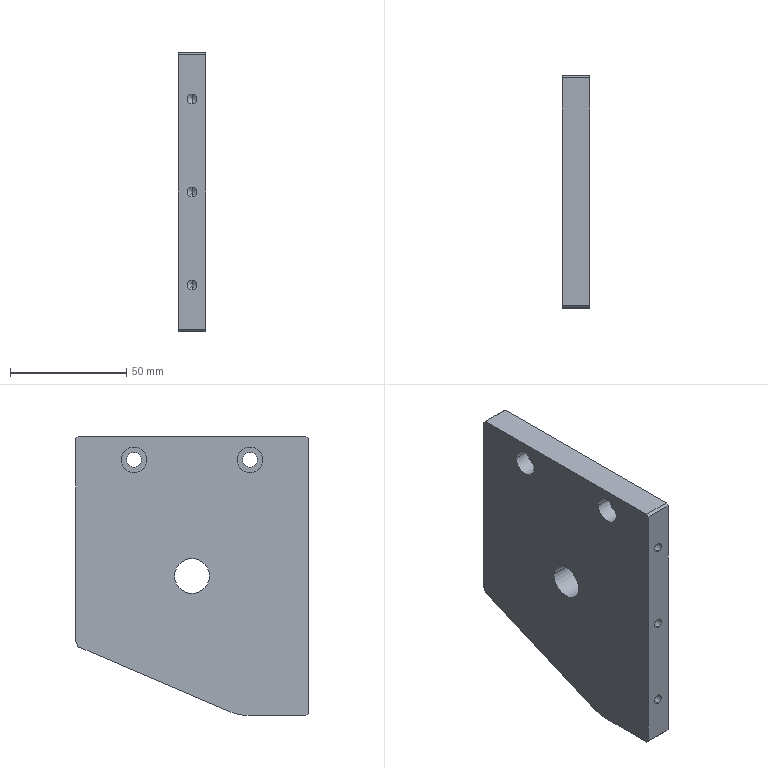Component | SolidWorks | V1ZHXTZ-AxisConnectionPlateReinforcementRibSB1-1 | 1 solid | 36 faces | box 12 x 100 x 120 mm | volume 126870 mm3 | cylinder 17 | plane 13 | cone 6 | commonest cylinder face diameters 4.2 x6 11 x4 6.4 x4 15 x2 40 x1
build123d program:
from build123d import *
from OCP.BRepFilletAPI import BRepFilletAPI_MakeChamfer

# Parameters (mm, degrees)
SKETCH1_W                                         = 120
SKETCH1_H                                         = 100
BOSS_EXTRUDE1_DEPTH                               = 6
CHAMFER1_SIZE                                     = 70
CHAMFER1_SIZE2                                    = 30
M5_TAPPED_HOLE2_D                                 = 4.2
M5_TAPPED_HOLE2_DEPTH                             = 17.4
M5_TAPPED_HOLE2_TIP                               = 1.262
HOLE_SIZE_ACCORDING_TO_TYPE_2_FOR_HEX_D           = 6.4
HOLE_SIZE_ACCORDING_TO_TYPE_2_FOR_HEX_DEPTH       = 18
HOLE_SIZE_ACCORDING_TO_TYPE_2_FOR_HEX_CBORE_D     = 11
HOLE_SIZE_ACCORDING_TO_TYPE_2_FOR_HEX_CBORE_DEPTH = 6.8
HOLE_SIZE_ACCORDING_TO_TYPE_2_FOR_HEX_TIP         = 1.923
CHAMFER2_SIZE                                     = 1
CHAMFER2_SIZE2                                    = 1.904
FILLET1_R                                         = 20
CUT_EXTRUDE1_REACH                                = 81.019
SKETCH10_R                                        = 7.5


with BuildPart() as part:
    # Sketch1 → Boss-Extrude1 (new, symmetric)
    with BuildSketch(Plane(origin=(0, 0, 0), x_dir=(1, 0, 0), z_dir=(0, 1, 0))):
        Rectangle(SKETCH1_W, SKETCH1_H)
    extrude(amount=BOSS_EXTRUDE1_DEPTH, both=True)

    # Chamfer1
    chamfer1_edges = [part.edges().sort_by_distance(p)[0] for p in [
        (-60, 0, 50),
    ]]
    chamfer1_side = [part.faces().sort_by_distance(p)[0] for p in [
        (-60, 0, 0),
    ]]
    chamfer(chamfer1_edges, length=CHAMFER1_SIZE, length2=CHAMFER1_SIZE2, reference=chamfer1_side[0])

    # M5 Tapped Hole2
    with Locations(Plane(origin=(0, 0, -50), x_dir=(-1, 0, 0), z_dir=(0, 0, -1))):
        with Locations((-40, 0), (40, 0), (0, 0)):
            Hole(M5_TAPPED_HOLE2_D / 2, depth=M5_TAPPED_HOLE2_DEPTH)
            with Locations((0, 0, -(M5_TAPPED_HOLE2_DEPTH + M5_TAPPED_HOLE2_TIP / 2))):  # 118° drill point
                Cone(0, M5_TAPPED_HOLE2_D / 2, M5_TAPPED_HOLE2_TIP, mode=Mode.SUBTRACT)

    # Hole Size _ according to_ Type 2 for Hex
    with Locations(Plane(origin=(0, -6, 0), x_dir=(-1, 0, 0), z_dir=(0, -1, 0))):
        with Locations((-50, 25), (-50, -25)):
            CounterBoreHole(HOLE_SIZE_ACCORDING_TO_TYPE_2_FOR_HEX_D / 2, HOLE_SIZE_ACCORDING_TO_TYPE_2_FOR_HEX_CBORE_D / 2, HOLE_SIZE_ACCORDING_TO_TYPE_2_FOR_HEX_CBORE_DEPTH, depth=HOLE_SIZE_ACCORDING_TO_TYPE_2_FOR_HEX_DEPTH)
            with Locations((0, 0, -(HOLE_SIZE_ACCORDING_TO_TYPE_2_FOR_HEX_DEPTH + HOLE_SIZE_ACCORDING_TO_TYPE_2_FOR_HEX_TIP / 2))):  # 118° drill point
                Cone(0, HOLE_SIZE_ACCORDING_TO_TYPE_2_FOR_HEX_D / 2, HOLE_SIZE_ACCORDING_TO_TYPE_2_FOR_HEX_TIP, mode=Mode.SUBTRACT)

    # Chamfer2: one chamfer whose edges measure the first distance from different faces: ONE call of the kernel's chamfer builder (chamfer() names one face for all edges)
    chamfer2_edges_1 = [part.edges().sort_by_distance(p)[0] for p in [
        (-30, 0, 50),
    ]]
    chamfer2_side_1 = [part.faces().sort_by_distance(p)[0] for p in [
        (-45, 0, 15),
    ]]
    chamfer2_edges_2 = [part.edges().sort_by_distance(p)[0] for p in [
        (60, 0, 50),
        (-60, 0, -50),
        (60, 0, -50),
    ]]
    chamfer2 = BRepFilletAPI_MakeChamfer(part.part.solid().wrapped)
    for e in chamfer2_edges_1:
        chamfer2.Add(CHAMFER2_SIZE, CHAMFER2_SIZE2, e.wrapped, chamfer2_side_1[0].wrapped)  # the first distance lies on this face
    for e in chamfer2_edges_2:
        chamfer2.Add(CHAMFER2_SIZE, e.wrapped)
    add(Compound.cast(chamfer2.Shape()), mode=Mode.REPLACE)

    # Fillet1
    fillet1_edges = [part.edges().sort_by_distance(p)[0] for p in [
        (-60, 0, -20),
    ]]
    fillet(fillet1_edges, radius=FILLET1_R)

    # Sketch10 → Cut-Extrude1 (cut, up to next)
    with BuildSketch(Plane.XZ.offset(6), mode=Mode.PRIVATE) as cut_extrude1_sk1:
        with Locations(Location((0, 0, 0), (0, 0, 270))):
            Circle(SKETCH10_R)
    cut_extrude1_tool1 = extrude(cut_extrude1_sk1.sketch, amount=-CUT_EXTRUDE1_REACH, mode=Mode.PRIVATE) & part.part
    add(cut_extrude1_tool1.solids().sort_by_distance((0, -6, 0))[0], mode=Mode.SUBTRACT)


solid = part.part

# Placed as in the assembly
solid = solid.moved(Location((105.521, -294.132, 508.739), (-90, 0, -90)))
STEP:
#1=CARTESIAN_POINT('',(4.391,-11.875,20.029));
#2=VERTEX_POINT('',#1);
#3=CARTESIAN_POINT('',(4.391,-11.285,20.029));
#4=VERTEX_POINT('',#3);
#5=CARTESIAN_POINT('',(4.391,-11.58,20.029));
#6=DIRECTION('',(1.,0.,-0.));
#7=DIRECTION('',(0.,-1.,-0.));
#8=AXIS2_PLACEMENT_3D('',#5,#6,#7);
#9=CIRCLE('',#8,0.2953);
#10=EDGE_CURVE('',#2,#4,#9,.T.);
#11=ORIENTED_EDGE('',*,*,#10,.T.);
#12=CARTESIAN_POINT('',(3.918,-11.285,20.029));
#13=VERTEX_POINT('',#12);
#14=CARTESIAN_POINT('',(4.391,-11.285,20.029));
#15=DIRECTION('',(-1.,-0.,0.));
#16=VECTOR('',#15,39.37);
#17=LINE('',#14,#16);
#18=EDGE_CURVE('',#4,#13,#17,.T.);
#19=ORIENTED_EDGE('',*,*,#18,.T.);
#20=CARTESIAN_POINT('',(3.918,-11.875,20.029));
#21=VERTEX_POINT('',#20);
#22=CARTESIAN_POINT('',(3.918,-11.58,20.029));
#23=DIRECTION('',(-1.,-0.,0.));
#24=DIRECTION('',(0.,-1.,-0.));
#25=AXIS2_PLACEMENT_3D('',#22,#23,#24);
#26=CIRCLE('',#25,0.2953);
#27=EDGE_CURVE('',#13,#21,#26,.T.);
#28=ORIENTED_EDGE('',*,*,#27,.T.);
#29=CARTESIAN_POINT('',(4.391,-11.875,20.029));
#30=DIRECTION('',(-1.,-0.,0.));
#31=VECTOR('',#30,39.37);
#32=LINE('',#29,#31);
#33=EDGE_CURVE('',#2,#21,#32,.T.);
#34=ORIENTED_EDGE('',*,*,#33,.F.);
#35=EDGE_LOOP('',(#11,#19,#28,#34));
#36=FACE_OUTER_BOUND('',#35,.T.);
#37=CARTESIAN_POINT('',(4.391,-11.58,20.029));
#38=DIRECTION('',(-1.,-0.,0.));
#39=DIRECTION('',(0.,-1.,-0.));
#40=AXIS2_PLACEMENT_3D('',#37,#38,#39);
#41=CYLINDRICAL_SURFACE('',#40,0.2953);
#42=ADVANCED_FACE('',(#36),#41,.F.);
#43=CARTESIAN_POINT('',(4.186,-12.348,21.998));
#44=VERTEX_POINT('',#43);
#45=CARTESIAN_POINT('',(4.186,-12.781,21.998));
#46=VERTEX_POINT('',#45);
#47=CARTESIAN_POINT('',(4.186,-12.564,21.998));
#48=DIRECTION('',(-1.,-0.,0.));
#49=DIRECTION('',(0.,-1.,-0.));
#50=AXIS2_PLACEMENT_3D('',#47,#48,#49);
#51=CIRCLE('',#50,0.2165);
#52=EDGE_CURVE('',#44,#46,#51,.T.);
#53=ORIENTED_EDGE('',*,*,#52,.F.);
#54=CARTESIAN_POINT('',(3.918,-12.348,21.998));
#55=VERTEX_POINT('',#54);
#56=CARTESIAN_POINT('',(3.918,-12.348,21.998));
#57=DIRECTION('',(-1.,-0.,0.));
#58=VECTOR('',#57,39.37);
#59=LINE('',#56,#58);
#60=EDGE_CURVE('',#44,#55,#59,.T.);
#61=ORIENTED_EDGE('',*,*,#60,.T.);
#62=CARTESIAN_POINT('',(3.918,-12.781,21.998));
#63=VERTEX_POINT('',#62);
#64=CARTESIAN_POINT('',(3.918,-12.564,21.998));
#65=DIRECTION('',(-1.,-0.,0.));
#66=DIRECTION('',(0.,-1.,-0.));
#67=AXIS2_PLACEMENT_3D('',#64,#65,#66);
#68=CIRCLE('',#67,0.2165);
#69=EDGE_CURVE('',#55,#63,#68,.T.);
#70=ORIENTED_EDGE('',*,*,#69,.T.);
#71=CARTESIAN_POINT('',(3.918,-12.781,21.998));
#72=DIRECTION('',(-1.,-0.,0.));
#73=VECTOR('',#72,39.37);
#74=LINE('',#71,#73);
#75=EDGE_CURVE('',#46,#63,#74,.T.);
#76=ORIENTED_EDGE('',*,*,#75,.F.);
#77=EDGE_LOOP('',(#53,#61,#70,#76));
#78=FACE_OUTER_BOUND('',#77,.T.);
#79=CARTESIAN_POINT('',(3.918,-12.564,21.998));
#80=DIRECTION('',(-1.,-0.,0.));
#81=DIRECTION('',(0.,-1.,-0.));
#82=AXIS2_PLACEMENT_3D('',#79,#80,#81);
#83=CYLINDRICAL_SURFACE('',#82,0.2165);
#84=ADVANCED_FACE('',(#78),#83,.F.);
#85=CARTESIAN_POINT('',(4.391,-12.438,21.998));
#86=VERTEX_POINT('',#85);
#87=CARTESIAN_POINT('',(4.391,-12.69,21.998));
#88=VERTEX_POINT('',#87);
#89=CARTESIAN_POINT('',(4.391,-12.564,21.998));
#90=DIRECTION('',(-1.,-0.,0.));
#91=DIRECTION('',(0.,-1.,-0.));
#92=AXIS2_PLACEMENT_3D('',#89,#90,#91);
#93=CIRCLE('',#92,0.126);
#94=EDGE_CURVE('',#86,#88,#93,.T.);
#95=ORIENTED_EDGE('',*,*,#94,.F.);
#96=CARTESIAN_POINT('',(4.186,-12.438,21.998));
#97=VERTEX_POINT('',#96);
#98=CARTESIAN_POINT('',(3.918,-12.438,21.998));
#99=DIRECTION('',(-1.,-0.,0.));
#100=VECTOR('',#99,39.37);
#101=LINE('',#98,#100);
#102=EDGE_CURVE('',#86,#97,#101,.T.);
#103=ORIENTED_EDGE('',*,*,#102,.T.);
#104=CARTESIAN_POINT('',(4.186,-12.69,21.998));
#105=VERTEX_POINT('',#104);
#106=CARTESIAN_POINT('',(4.186,-12.564,21.998));
#107=DIRECTION('',(-1.,-0.,0.));
#108=DIRECTION('',(0.,-1.,-0.));
#109=AXIS2_PLACEMENT_3D('',#106,#107,#108);
#110=CIRCLE('',#109,0.126);
#111=EDGE_CURVE('',#97,#105,#110,.T.);
#112=ORIENTED_EDGE('',*,*,#111,.T.);
#113=CARTESIAN_POINT('',(3.918,-12.69,21.998));
#114=DIRECTION('',(-1.,-0.,0.));
#115=VECTOR('',#114,39.37);
#116=LINE('',#113,#115);
#117=EDGE_CURVE('',#88,#105,#116,.T.);
#118=ORIENTED_EDGE('',*,*,#117,.F.);
#119=EDGE_LOOP('',(#95,#103,#112,#118));
#120=FACE_OUTER_BOUND('',#119,.T.);
#121=CARTESIAN_POINT('',(3.918,-12.564,21.998));
#122=DIRECTION('',(-1.,-0.,0.));
#123=DIRECTION('',(0.,-1.,-0.));
#124=AXIS2_PLACEMENT_3D('',#121,#122,#123);
#125=CYLINDRICAL_SURFACE('',#124,0.126);
#126=ADVANCED_FACE('',(#120),#125,.F.);
#127=CARTESIAN_POINT('',(4.186,-10.379,21.998));
#128=VERTEX_POINT('',#127);
#129=CARTESIAN_POINT('',(4.186,-10.812,21.998));
#130=VERTEX_POINT('',#129);
#131=CARTESIAN_POINT('',(4.186,-10.596,21.998));
#132=DIRECTION('',(-1.,-0.,0.));
#133=DIRECTION('',(0.,-1.,-0.));
#134=AXIS2_PLACEMENT_3D('',#131,#132,#133);
#135=CIRCLE('',#134,0.2165);
#136=EDGE_CURVE('',#128,#130,#135,.T.);
#137=ORIENTED_EDGE('',*,*,#136,.F.);
#138=CARTESIAN_POINT('',(3.918,-10.379,21.998));
#139=VERTEX_POINT('',#138);
#140=CARTESIAN_POINT('',(3.918,-10.379,21.998));
#141=DIRECTION('',(-1.,-0.,0.));
#142=VECTOR('',#141,39.37);
#143=LINE('',#140,#142);
#144=EDGE_CURVE('',#128,#139,#143,.T.);
#145=ORIENTED_EDGE('',*,*,#144,.T.);
#146=CARTESIAN_POINT('',(3.918,-10.812,21.998));
#147=VERTEX_POINT('',#146);
#148=CARTESIAN_POINT('',(3.918,-10.596,21.998));
#149=DIRECTION('',(-1.,-0.,0.));
#150=DIRECTION('',(0.,-1.,-0.));
#151=AXIS2_PLACEMENT_3D('',#148,#149,#150);
#152=CIRCLE('',#151,0.2165);
#153=EDGE_CURVE('',#139,#147,#152,.T.);
#154=ORIENTED_EDGE('',*,*,#153,.T.);
#155=CARTESIAN_POINT('',(3.918,-10.812,21.998));
#156=DIRECTION('',(-1.,-0.,0.));
#157=VECTOR('',#156,39.37);
#158=LINE('',#155,#157);
#159=EDGE_CURVE('',#130,#147,#158,.T.);
#160=ORIENTED_EDGE('',*,*,#159,.F.);
#161=EDGE_LOOP('',(#137,#145,#154,#160));
#162=FACE_OUTER_BOUND('',#161,.T.);
#163=CARTESIAN_POINT('',(3.918,-10.596,21.998));
#164=DIRECTION('',(-1.,-0.,0.));
#165=DIRECTION('',(0.,-1.,-0.));
#166=AXIS2_PLACEMENT_3D('',#163,#164,#165);
#167=CYLINDRICAL_SURFACE('',#166,0.2165);
#168=ADVANCED_FACE('',(#162),#167,.F.);
#169=CARTESIAN_POINT('',(4.391,-10.47,21.998));
#170=VERTEX_POINT('',#169);
#171=CARTESIAN_POINT('',(4.391,-10.722,21.998));
#172=VERTEX_POINT('',#171);
#173=CARTESIAN_POINT('',(4.391,-10.596,21.998));
#174=DIRECTION('',(-1.,-0.,0.));
#175=DIRECTION('',(0.,-1.,-0.));
#176=AXIS2_PLACEMENT_3D('',#173,#174,#175);
#177=CIRCLE('',#176,0.126);
#178=EDGE_CURVE('',#170,#172,#177,.T.);
#179=ORIENTED_EDGE('',*,*,#178,.F.);
#180=CARTESIAN_POINT('',(4.186,-10.47,21.998));
#181=VERTEX_POINT('',#180);
#182=CARTESIAN_POINT('',(3.918,-10.47,21.998));
#183=DIRECTION('',(-1.,-0.,0.));
#184=VECTOR('',#183,39.37);
#185=LINE('',#182,#184);
#186=EDGE_CURVE('',#170,#181,#185,.T.);
#187=ORIENTED_EDGE('',*,*,#186,.T.);
#188=CARTESIAN_POINT('',(4.186,-10.722,21.998));
#189=VERTEX_POINT('',#188);
#190=CARTESIAN_POINT('',(4.186,-10.596,21.998));
#191=DIRECTION('',(-1.,-0.,0.));
#192=DIRECTION('',(0.,-1.,-0.));
#193=AXIS2_PLACEMENT_3D('',#190,#191,#192);
#194=CIRCLE('',#193,0.126);
#195=EDGE_CURVE('',#181,#189,#194,.T.);
#196=ORIENTED_EDGE('',*,*,#195,.T.);
#197=CARTESIAN_POINT('',(3.918,-10.722,21.998));
#198=DIRECTION('',(-1.,-0.,0.));
#199=VECTOR('',#198,39.37);
#200=LINE('',#197,#199);
#201=EDGE_CURVE('',#172,#189,#200,.T.);
#202=ORIENTED_EDGE('',*,*,#201,.F.);
#203=EDGE_LOOP('',(#179,#187,#196,#202));
#204=FACE_OUTER_BOUND('',#203,.T.);
#205=CARTESIAN_POINT('',(3.918,-10.596,21.998));
#206=DIRECTION('',(-1.,-0.,0.));
#207=DIRECTION('',(0.,-1.,-0.));
#208=AXIS2_PLACEMENT_3D('',#205,#206,#207);
#209=CYLINDRICAL_SURFACE('',#208,0.126);
#210=ADVANCED_FACE('',(#204),#209,.F.);
#211=CARTESIAN_POINT('',(4.154,-12.863,21.687));
#212=VERTEX_POINT('',#211);
#213=CARTESIAN_POINT('',(4.154,-12.863,21.521));
#214=VERTEX_POINT('',#213);
#215=CARTESIAN_POINT('',(4.154,-12.863,21.604));
#216=DIRECTION('',(0.,-1.,-0.));
#217=DIRECTION('',(0.,0.,-1.));
#218=AXIS2_PLACEMENT_3D('',#215,#216,#217);
#219=CIRCLE('',#218,0.08268);
#220=EDGE_CURVE('',#212,#214,#219,.T.);
#221=ORIENTED_EDGE('',*,*,#220,.F.);
#222=CARTESIAN_POINT('',(4.154,-13.548,21.687));
#223=VERTEX_POINT('',#222);
#224=CARTESIAN_POINT('',(4.154,-13.548,21.687));
#225=DIRECTION('',(0.,-1.,-0.));
#226=VECTOR('',#225,39.37);
#227=LINE('',#224,#226);
#228=EDGE_CURVE('',#212,#223,#227,.T.);
#229=ORIENTED_EDGE('',*,*,#228,.T.);
#230=CARTESIAN_POINT('',(4.154,-13.548,21.521));
#231=VERTEX_POINT('',#230);
#232=CARTESIAN_POINT('',(4.154,-13.548,21.604));
#233=DIRECTION('',(0.,-1.,-0.));
#234=DIRECTION('',(0.,0.,-1.));
#235=AXIS2_PLACEMENT_3D('',#232,#233,#234);
#236=CIRCLE('',#235,0.08268);
#237=EDGE_CURVE('',#223,#231,#236,.T.);
#238=ORIENTED_EDGE('',*,*,#237,.T.);
#239=CARTESIAN_POINT('',(4.154,-13.548,21.521));
#240=DIRECTION('',(0.,-1.,-0.));
#241=VECTOR('',#240,39.37);
#242=LINE('',#239,#241);
#243=EDGE_CURVE('',#214,#231,#242,.T.);
#244=ORIENTED_EDGE('',*,*,#243,.F.);
#245=EDGE_LOOP('',(#221,#229,#238,#244));
#246=FACE_OUTER_BOUND('',#245,.T.);
#247=CARTESIAN_POINT('',(4.154,-13.548,21.604));
#248=DIRECTION('',(0.,-1.,-0.));
#249=DIRECTION('',(0.,0.,-1.));
#250=AXIS2_PLACEMENT_3D('',#247,#248,#249);
#251=CYLINDRICAL_SURFACE('',#250,0.08268);
#252=ADVANCED_FACE('',(#246),#251,.F.);
#253=CARTESIAN_POINT('',(4.154,-12.814,21.604));
#254=VERTEX_POINT('',#253);
#255=CARTESIAN_POINT('',(4.154,-12.863,21.521));
#256=DIRECTION('',(0.,-0.515,-0.8572));
#257=VECTOR('',#256,39.37);
#258=LINE('',#255,#257);
#259=EDGE_CURVE('',#254,#214,#258,.T.);
#260=ORIENTED_EDGE('',*,*,#259,.F.);
#261=CARTESIAN_POINT('',(4.154,-12.863,21.687));
#262=DIRECTION('',(0.,-0.515,0.8572));
#263=VECTOR('',#262,39.37);
#264=LINE('',#261,#263);
#265=EDGE_CURVE('',#254,#212,#264,.T.);
#266=ORIENTED_EDGE('',*,*,#265,.T.);
#267=ORIENTED_EDGE('',*,*,#220,.T.);
#268=EDGE_LOOP('',(#260,#266,#267));
#269=FACE_OUTER_BOUND('',#268,.T.);
#270=CARTESIAN_POINT('',(4.154,-12.863,21.604));
#271=DIRECTION('',(0.,-1.,-0.));
#272=DIRECTION('',(0.,0.,-1.));
#273=AXIS2_PLACEMENT_3D('',#270,#271,#272);
#274=CONICAL_SURFACE('',#273,0.08268,1.03);
#275=ADVANCED_FACE('',(#269),#274,.F.);
#276=CARTESIAN_POINT('',(4.154,-12.863,18.537));
#277=VERTEX_POINT('',#276);
#278=CARTESIAN_POINT('',(4.154,-12.863,18.372));
#279=VERTEX_POINT('',#278);
#280=CARTESIAN_POINT('',(4.154,-12.863,18.454));
#281=DIRECTION('',(0.,-1.,-0.));
#282=DIRECTION('',(0.,0.,-1.));
#283=AXIS2_PLACEMENT_3D('',#280,#281,#282);
#284=CIRCLE('',#283,0.08268);
#285=EDGE_CURVE('',#277,#279,#284,.T.);
#286=ORIENTED_EDGE('',*,*,#285,.F.);
#287=CARTESIAN_POINT('',(4.154,-13.548,18.537));
#288=VERTEX_POINT('',#287);
#289=CARTESIAN_POINT('',(4.154,-13.548,18.537));
#290=DIRECTION('',(0.,-1.,-0.));
#291=VECTOR('',#290,39.37);
#292=LINE('',#289,#291);
#293=EDGE_CURVE('',#277,#288,#292,.T.);
#294=ORIENTED_EDGE('',*,*,#293,.T.);
#295=CARTESIAN_POINT('',(4.154,-13.548,18.372));
#296=VERTEX_POINT('',#295);
#297=CARTESIAN_POINT('',(4.154,-13.548,18.454));
#298=DIRECTION('',(0.,-1.,-0.));
#299=DIRECTION('',(0.,0.,-1.));
#300=AXIS2_PLACEMENT_3D('',#297,#298,#299);
#301=CIRCLE('',#300,0.08268);
#302=EDGE_CURVE('',#288,#296,#301,.T.);
#303=ORIENTED_EDGE('',*,*,#302,.T.);
#304=CARTESIAN_POINT('',(4.154,-13.548,18.372));
#305=DIRECTION('',(0.,-1.,-0.));
#306=VECTOR('',#305,39.37);
#307=LINE('',#304,#306);
#308=EDGE_CURVE('',#279,#296,#307,.T.);
#309=ORIENTED_EDGE('',*,*,#308,.F.);
#310=EDGE_LOOP('',(#286,#294,#303,#309));
#311=FACE_OUTER_BOUND('',#310,.T.);
#312=CARTESIAN_POINT('',(4.154,-13.548,18.454));
#313=DIRECTION('',(0.,-1.,-0.));
#314=DIRECTION('',(0.,0.,-1.));
#315=AXIS2_PLACEMENT_3D('',#312,#313,#314);
#316=CYLINDRICAL_SURFACE('',#315,0.08268);
#317=ADVANCED_FACE('',(#311),#316,.F.);
#318=CARTESIAN_POINT('',(4.154,-12.814,18.454));
#319=VERTEX_POINT('',#318);
#320=CARTESIAN_POINT('',(4.154,-12.863,18.372));
#321=DIRECTION('',(0.,-0.515,-0.8572));
#322=VECTOR('',#321,39.37);
#323=LINE('',#320,#322);
#324=EDGE_CURVE('',#319,#279,#323,.T.);
#325=ORIENTED_EDGE('',*,*,#324,.F.);
#326=CARTESIAN_POINT('',(4.154,-12.863,18.537));
#327=DIRECTION('',(0.,-0.515,0.8572));
#328=VECTOR('',#327,39.37);
#329=LINE('',#326,#328);
#330=EDGE_CURVE('',#319,#277,#329,.T.);
#331=ORIENTED_EDGE('',*,*,#330,.T.);
#332=ORIENTED_EDGE('',*,*,#285,.T.);
#333=EDGE_LOOP('',(#325,#331,#332));
#334=FACE_OUTER_BOUND('',#333,.T.);
#335=CARTESIAN_POINT('',(4.154,-12.863,18.454));
#336=DIRECTION('',(0.,-1.,-0.));
#337=DIRECTION('',(0.,0.,-1.));
#338=AXIS2_PLACEMENT_3D('',#335,#336,#337);
#339=CONICAL_SURFACE('',#338,0.08268,1.03);
#340=ADVANCED_FACE('',(#334),#339,.F.);
#341=CARTESIAN_POINT('',(4.154,-12.863,20.112));
#342=VERTEX_POINT('',#341);
#343=CARTESIAN_POINT('',(4.154,-12.863,19.946));
#344=VERTEX_POINT('',#343);
#345=CARTESIAN_POINT('',(4.154,-12.863,20.029));
#346=DIRECTION('',(0.,-1.,-0.));
#347=DIRECTION('',(0.,0.,-1.));
#348=AXIS2_PLACEMENT_3D('',#345,#346,#347);
#349=CIRCLE('',#348,0.08268);
#350=EDGE_CURVE('',#342,#344,#349,.T.);
#351=ORIENTED_EDGE('',*,*,#350,.F.);
#352=CARTESIAN_POINT('',(4.154,-13.548,20.112));
#353=VERTEX_POINT('',#352);
#354=CARTESIAN_POINT('',(4.154,-13.548,20.112));
#355=DIRECTION('',(0.,-1.,-0.));
#356=VECTOR('',#355,39.37);
#357=LINE('',#354,#356);
#358=EDGE_CURVE('',#342,#353,#357,.T.);
#359=ORIENTED_EDGE('',*,*,#358,.T.);
#360=CARTESIAN_POINT('',(4.154,-13.548,19.946));
#361=VERTEX_POINT('',#360);
#362=CARTESIAN_POINT('',(4.154,-13.548,20.029));
#363=DIRECTION('',(0.,-1.,-0.));
#364=DIRECTION('',(0.,0.,-1.));
#365=AXIS2_PLACEMENT_3D('',#362,#363,#364);
#366=CIRCLE('',#365,0.08268);
#367=EDGE_CURVE('',#353,#361,#366,.T.);
#368=ORIENTED_EDGE('',*,*,#367,.T.);
#369=CARTESIAN_POINT('',(4.154,-13.548,19.946));
#370=DIRECTION('',(0.,-1.,-0.));
#371=VECTOR('',#370,39.37);
#372=LINE('',#369,#371);
#373=EDGE_CURVE('',#344,#361,#372,.T.);
#374=ORIENTED_EDGE('',*,*,#373,.F.);
#375=EDGE_LOOP('',(#351,#359,#368,#374));
#376=FACE_OUTER_BOUND('',#375,.T.);
#377=CARTESIAN_POINT('',(4.154,-13.548,20.029));
#378=DIRECTION('',(0.,-1.,-0.));
#379=DIRECTION('',(0.,0.,-1.));
#380=AXIS2_PLACEMENT_3D('',#377,#378,#379);
#381=CYLINDRICAL_SURFACE('',#380,0.08268);
#382=ADVANCED_FACE('',(#376),#381,.F.);
#383=CARTESIAN_POINT('',(4.154,-12.814,20.029));
#384=VERTEX_POINT('',#383);
#385=CARTESIAN_POINT('',(4.154,-12.863,19.946));
#386=DIRECTION('',(0.,-0.515,-0.8572));
#387=VECTOR('',#386,39.37);
#388=LINE('',#385,#387);
#389=EDGE_CURVE('',#384,#344,#388,.T.);
#390=ORIENTED_EDGE('',*,*,#389,.F.);
#391=CARTESIAN_POINT('',(4.154,-12.863,20.112));
#392=DIRECTION('',(0.,-0.515,0.8572));
#393=VECTOR('',#392,39.37);
#394=LINE('',#391,#393);
#395=EDGE_CURVE('',#384,#342,#394,.T.);
#396=ORIENTED_EDGE('',*,*,#395,.T.);
#397=ORIENTED_EDGE('',*,*,#350,.T.);
#398=EDGE_LOOP('',(#390,#396,#397));
#399=FACE_OUTER_BOUND('',#398,.T.);
#400=CARTESIAN_POINT('',(4.154,-12.863,20.029));
#401=DIRECTION('',(0.,-1.,-0.));
#402=DIRECTION('',(0.,0.,-1.));
#403=AXIS2_PLACEMENT_3D('',#400,#401,#402);
#404=CONICAL_SURFACE('',#403,0.08268,1.03);
#405=ADVANCED_FACE('',(#399),#404,.F.);
#406=CARTESIAN_POINT('',(4.391,-9.651,22.391));
#407=VERTEX_POINT('',#406);
#408=CARTESIAN_POINT('',(4.391,-13.509,22.391));
#409=VERTEX_POINT('',#408);
#410=CARTESIAN_POINT('',(4.391,-9.611,22.391));
#411=DIRECTION('',(0.,-1.,-0.));
#412=VECTOR('',#411,39.37);
#413=LINE('',#410,#412);
#414=EDGE_CURVE('',#407,#409,#413,.T.);
#415=ORIENTED_EDGE('',*,*,#414,.F.);
#416=CARTESIAN_POINT('',(3.918,-9.651,22.391));
#417=VERTEX_POINT('',#416);
#418=CARTESIAN_POINT('',(4.391,-9.651,22.391));
#419=DIRECTION('',(-1.,-0.,0.));
#420=VECTOR('',#419,39.37);
#421=LINE('',#418,#420);
#422=EDGE_CURVE('',#407,#417,#421,.T.);
#423=ORIENTED_EDGE('',*,*,#422,.T.);
#424=CARTESIAN_POINT('',(3.918,-13.509,22.391));
#425=VERTEX_POINT('',#424);
#426=CARTESIAN_POINT('',(3.918,-9.611,22.391));
#427=DIRECTION('',(0.,-1.,-0.));
#428=VECTOR('',#427,39.37);
#429=LINE('',#426,#428);
#430=EDGE_CURVE('',#417,#425,#429,.T.);
#431=ORIENTED_EDGE('',*,*,#430,.T.);
#432=CARTESIAN_POINT('',(4.391,-13.509,22.391));
#433=DIRECTION('',(1.,0.,-0.));
#434=VECTOR('',#433,39.37);
#435=LINE('',#432,#434);
#436=EDGE_CURVE('',#425,#409,#435,.T.);
#437=ORIENTED_EDGE('',*,*,#436,.T.);
#438=EDGE_LOOP('',(#415,#423,#431,#437));
#439=FACE_OUTER_BOUND('',#438,.T.);
#440=CARTESIAN_POINT('',(4.391,-9.611,22.391));
#441=DIRECTION('',(-0.,0.,-1.));
#442=DIRECTION('',(-0.,1.,0.));
#443=AXIS2_PLACEMENT_3D('',#440,#441,#442);
#444=PLANE('',#443);
#445=ADVANCED_FACE('',(#439),#444,.F.);
#446=CARTESIAN_POINT('',(4.154,-13.548,21.604));
#447=DIRECTION('',(0.,-1.,-0.));
#448=DIRECTION('',(0.,0.,-1.));
#449=AXIS2_PLACEMENT_3D('',#446,#447,#448);
#450=CIRCLE('',#449,0.08268);
#451=EDGE_CURVE('',#231,#223,#450,.T.);
#452=ORIENTED_EDGE('',*,*,#451,.F.);
#453=ORIENTED_EDGE('',*,*,#237,.F.);
#454=EDGE_LOOP('',(#452,#453));
#455=FACE_BOUND('',#454,.T.);
#456=CARTESIAN_POINT('',(4.154,-13.548,18.454));
#457=DIRECTION('',(0.,-1.,-0.));
#458=DIRECTION('',(0.,0.,-1.));
#459=AXIS2_PLACEMENT_3D('',#456,#457,#458);
#460=CIRCLE('',#459,0.08268);
#461=EDGE_CURVE('',#296,#288,#460,.T.);
#462=ORIENTED_EDGE('',*,*,#461,.F.);
#463=ORIENTED_EDGE('',*,*,#302,.F.);
#464=EDGE_LOOP('',(#462,#463));
#465=FACE_BOUND('',#464,.T.);
#466=CARTESIAN_POINT('',(4.154,-13.548,20.029));
#467=DIRECTION('',(0.,-1.,-0.));
#468=DIRECTION('',(0.,0.,-1.));
#469=AXIS2_PLACEMENT_3D('',#466,#467,#468);
#470=CIRCLE('',#469,0.08268);
#471=EDGE_CURVE('',#361,#353,#470,.T.);
#472=ORIENTED_EDGE('',*,*,#471,.F.);
#473=ORIENTED_EDGE('',*,*,#367,.F.);
#474=EDGE_LOOP('',(#472,#473));
#475=FACE_BOUND('',#474,.T.);
#476=CARTESIAN_POINT('',(4.391,-13.548,22.352));
#477=VERTEX_POINT('',#476);
#478=CARTESIAN_POINT('',(4.391,-13.548,17.706));
#479=VERTEX_POINT('',#478);
#480=CARTESIAN_POINT('',(4.391,-13.548,17.667));
#481=DIRECTION('',(-0.,0.,-1.));
#482=VECTOR('',#481,39.37);
#483=LINE('',#480,#482);
#484=EDGE_CURVE('',#477,#479,#483,.T.);
#485=ORIENTED_EDGE('',*,*,#484,.F.);
#486=CARTESIAN_POINT('',(3.918,-13.548,22.352));
#487=VERTEX_POINT('',#486);
#488=CARTESIAN_POINT('',(4.391,-13.548,22.352));
#489=DIRECTION('',(-1.,-0.,0.));
#490=VECTOR('',#489,39.37);
#491=LINE('',#488,#490);
#492=EDGE_CURVE('',#477,#487,#491,.T.);
#493=ORIENTED_EDGE('',*,*,#492,.T.);
#494=CARTESIAN_POINT('',(3.918,-13.548,17.706));
#495=VERTEX_POINT('',#494);
#496=CARTESIAN_POINT('',(3.918,-13.548,17.667));
#497=DIRECTION('',(-0.,0.,-1.));
#498=VECTOR('',#497,39.37);
#499=LINE('',#496,#498);
#500=EDGE_CURVE('',#487,#495,#499,.T.);
#501=ORIENTED_EDGE('',*,*,#500,.T.);
#502=CARTESIAN_POINT('',(4.391,-13.548,17.706));
#503=DIRECTION('',(1.,0.,-0.));
#504=VECTOR('',#503,39.37);
#505=LINE('',#502,#504);
#506=EDGE_CURVE('',#495,#479,#505,.T.);
#507=ORIENTED_EDGE('',*,*,#506,.T.);
#508=EDGE_LOOP('',(#485,#493,#501,#507));
#509=FACE_OUTER_BOUND('',#508,.T.);
#510=CARTESIAN_POINT('',(4.391,-13.548,17.667));
#511=DIRECTION('',(-0.,1.,0.));
#512=DIRECTION('',(0.,-0.,1.));
#513=AXIS2_PLACEMENT_3D('',#510,#511,#512);
#514=PLANE('',#513);
#515=ADVANCED_FACE('',(#455,#465,#475,#509),#514,.F.);
#516=CARTESIAN_POINT('',(3.918,-13.509,17.667));
#517=VERTEX_POINT('',#516);
#518=CARTESIAN_POINT('',(3.918,-12.529,17.667));
#519=VERTEX_POINT('',#518);
#520=CARTESIAN_POINT('',(3.918,-9.611,17.667));
#521=DIRECTION('',(-0.,1.,0.));
#522=VECTOR('',#521,39.37);
#523=LINE('',#520,#522);
#524=EDGE_CURVE('',#517,#519,#523,.T.);
#525=ORIENTED_EDGE('',*,*,#524,.T.);
#526=CARTESIAN_POINT('',(4.391,-12.529,17.667));
#527=VERTEX_POINT('',#526);
#528=CARTESIAN_POINT('',(4.391,-12.529,17.667));
#529=DIRECTION('',(1.,0.,-0.));
#530=VECTOR('',#529,39.37);
#531=LINE('',#528,#530);
#532=EDGE_CURVE('',#519,#527,#531,.T.);
#533=ORIENTED_EDGE('',*,*,#532,.T.);
#534=CARTESIAN_POINT('',(4.391,-13.509,17.667));
#535=VERTEX_POINT('',#534);
#536=CARTESIAN_POINT('',(4.391,-9.611,17.667));
#537=DIRECTION('',(-0.,1.,0.));
#538=VECTOR('',#537,39.37);
#539=LINE('',#536,#538);
#540=EDGE_CURVE('',#535,#527,#539,.T.);
#541=ORIENTED_EDGE('',*,*,#540,.F.);
#542=CARTESIAN_POINT('',(4.391,-13.509,17.667));
#543=DIRECTION('',(-1.,-0.,0.));
#544=VECTOR('',#543,39.37);
#545=LINE('',#542,#544);
#546=EDGE_CURVE('',#535,#517,#545,.T.);
#547=ORIENTED_EDGE('',*,*,#546,.T.);
#548=EDGE_LOOP('',(#525,#533,#541,#547));
#549=FACE_OUTER_BOUND('',#548,.T.);
#550=CARTESIAN_POINT('',(4.391,-9.611,17.667));
#551=DIRECTION('',(0.,-0.,1.));
#552=DIRECTION('',(0.,-1.,-0.));
#553=AXIS2_PLACEMENT_3D('',#550,#551,#552);
#554=PLANE('',#553);
#555=ADVANCED_FACE('',(#549),#554,.F.);
#556=CARTESIAN_POINT('',(4.391,-9.611,18.923));
#557=VERTEX_POINT('',#556);
#558=CARTESIAN_POINT('',(4.391,-9.611,22.352));
#559=VERTEX_POINT('',#558);
#560=CARTESIAN_POINT('',(4.391,-9.611,17.667));
#561=DIRECTION('',(0.,-0.,1.));
#562=VECTOR('',#561,39.37);
#563=LINE('',#560,#562);
#564=EDGE_CURVE('',#557,#559,#563,.T.);
#565=ORIENTED_EDGE('',*,*,#564,.F.);
#566=CARTESIAN_POINT('',(3.918,-9.611,18.923));
#567=VERTEX_POINT('',#566);
#568=CARTESIAN_POINT('',(3.918,-9.611,18.923));
#569=DIRECTION('',(-1.,-0.,0.));
#570=VECTOR('',#569,39.37);
#571=LINE('',#568,#570);
#572=EDGE_CURVE('',#557,#567,#571,.T.);
#573=ORIENTED_EDGE('',*,*,#572,.T.);
#574=CARTESIAN_POINT('',(3.918,-9.611,22.352));
#575=VERTEX_POINT('',#574);
#576=CARTESIAN_POINT('',(3.918,-9.611,17.667));
#577=DIRECTION('',(0.,-0.,1.));
#578=VECTOR('',#577,39.37);
#579=LINE('',#576,#578);
#580=EDGE_CURVE('',#567,#575,#579,.T.);
#581=ORIENTED_EDGE('',*,*,#580,.T.);
#582=CARTESIAN_POINT('',(4.391,-9.611,22.352));
#583=DIRECTION('',(1.,0.,-0.));
#584=VECTOR('',#583,39.37);
#585=LINE('',#582,#584);
#586=EDGE_CURVE('',#575,#559,#585,.T.);
#587=ORIENTED_EDGE('',*,*,#586,.T.);
#588=EDGE_LOOP('',(#565,#573,#581,#587));
#589=FACE_OUTER_BOUND('',#588,.T.);
#590=CARTESIAN_POINT('',(4.391,-9.611,17.667));
#591=DIRECTION('',(0.,-1.,-0.));
#592=DIRECTION('',(-0.,0.,-1.));
#593=AXIS2_PLACEMENT_3D('',#590,#591,#592);
#594=PLANE('',#593);
#595=ADVANCED_FACE('',(#589),#594,.F.);
#596=ORIENTED_EDGE('',*,*,#10,.F.);
#597=CARTESIAN_POINT('',(4.391,-11.58,20.029));
#598=DIRECTION('',(1.,0.,-0.));
#599=DIRECTION('',(0.,-1.,-0.));
#600=AXIS2_PLACEMENT_3D('',#597,#598,#599);
#601=CIRCLE('',#600,0.2953);
#602=EDGE_CURVE('',#4,#2,#601,.T.);
#603=ORIENTED_EDGE('',*,*,#602,.F.);
#604=EDGE_LOOP('',(#596,#603));
#605=FACE_BOUND('',#604,.T.);
#606=CARTESIAN_POINT('',(4.391,-12.564,21.998));
#607=DIRECTION('',(-1.,-0.,0.));
#608=DIRECTION('',(0.,-1.,-0.));
#609=AXIS2_PLACEMENT_3D('',#606,#607,#608);
#610=CIRCLE('',#609,0.126);
#611=EDGE_CURVE('',#88,#86,#610,.T.);
#612=ORIENTED_EDGE('',*,*,#611,.T.);
#613=ORIENTED_EDGE('',*,*,#94,.T.);
#614=EDGE_LOOP('',(#612,#613));
#615=FACE_BOUND('',#614,.T.);
#616=CARTESIAN_POINT('',(4.391,-10.596,21.998));
#617=DIRECTION('',(-1.,-0.,0.));
#618=DIRECTION('',(0.,-1.,-0.));
#619=AXIS2_PLACEMENT_3D('',#616,#617,#618);
#620=CIRCLE('',#619,0.126);
#621=EDGE_CURVE('',#172,#170,#620,.T.);
#622=ORIENTED_EDGE('',*,*,#621,.T.);
#623=ORIENTED_EDGE('',*,*,#178,.T.);
#624=EDGE_LOOP('',(#622,#623));
#625=FACE_BOUND('',#624,.T.);
#626=ORIENTED_EDGE('',*,*,#540,.T.);
#627=CARTESIAN_POINT('',(4.391,-12.219,17.731));
#628=VERTEX_POINT('',#627);
#629=CARTESIAN_POINT('',(4.391,-12.529,18.454));
#630=DIRECTION('',(1.,0.,-0.));
#631=DIRECTION('',(0.,-1.,-0.));
#632=AXIS2_PLACEMENT_3D('',#629,#630,#631);
#633=CIRCLE('',#632,0.7874);
#634=EDGE_CURVE('',#527,#628,#633,.T.);
#635=ORIENTED_EDGE('',*,*,#634,.T.);
#636=CARTESIAN_POINT('',(4.391,-9.648,18.832));
#637=VERTEX_POINT('',#636);
#638=CARTESIAN_POINT('',(4.391,-9.611,18.848));
#639=DIRECTION('',(-0.,0.9191,0.3939));
#640=VECTOR('',#639,39.37);
#641=LINE('',#638,#640);
#642=EDGE_CURVE('',#628,#637,#641,.T.);
#643=ORIENTED_EDGE('',*,*,#642,.T.);
#644=CARTESIAN_POINT('',(4.391,-9.611,18.923));
#645=DIRECTION('',(-0.,0.3714,0.9285));
#646=VECTOR('',#645,39.37);
#647=LINE('',#644,#646);
#648=EDGE_CURVE('',#637,#557,#647,.T.);
#649=ORIENTED_EDGE('',*,*,#648,.T.);
#650=ORIENTED_EDGE('',*,*,#564,.T.);
#651=CARTESIAN_POINT('',(4.391,-9.651,22.391));
#652=DIRECTION('',(0.,-0.7071,0.7071));
#653=VECTOR('',#652,39.37);
#654=LINE('',#651,#653);
#655=EDGE_CURVE('',#559,#407,#654,.T.);
#656=ORIENTED_EDGE('',*,*,#655,.T.);
#657=ORIENTED_EDGE('',*,*,#414,.T.);
#658=CARTESIAN_POINT('',(4.391,-13.548,22.352));
#659=DIRECTION('',(0.,-0.7071,-0.7071));
#660=VECTOR('',#659,39.37);
#661=LINE('',#658,#660);
#662=EDGE_CURVE('',#409,#477,#661,.T.);
#663=ORIENTED_EDGE('',*,*,#662,.T.);
#664=ORIENTED_EDGE('',*,*,#484,.T.);
#665=CARTESIAN_POINT('',(4.391,-13.509,17.667));
#666=DIRECTION('',(-0.,0.7071,-0.7071));
#667=VECTOR('',#666,39.37);
#668=LINE('',#665,#667);
#669=EDGE_CURVE('',#479,#535,#668,.T.);
#670=ORIENTED_EDGE('',*,*,#669,.T.);
#671=EDGE_LOOP('',(#626,#635,#643,#649,#650,#656,#657,#663,#664,#670));
#672=FACE_OUTER_BOUND('',#671,.T.);
#673=CARTESIAN_POINT('',(4.391,-11.58,20.029));
#674=DIRECTION('',(-1.,-0.,0.));
#675=DIRECTION('',(0.,-1.,-0.));
#676=AXIS2_PLACEMENT_3D('',#673,#674,#675);
#677=PLANE('',#676);
#678=ADVANCED_FACE('',(#605,#615,#625,#672),#677,.F.);
#679=CARTESIAN_POINT('',(3.918,-11.58,20.029));
#680=DIRECTION('',(-1.,-0.,0.));
#681=DIRECTION('',(0.,-1.,-0.));
#682=AXIS2_PLACEMENT_3D('',#679,#680,#681);
#683=CIRCLE('',#682,0.2953);
#684=EDGE_CURVE('',#21,#13,#683,.T.);
#685=ORIENTED_EDGE('',*,*,#684,.F.);
#686=ORIENTED_EDGE('',*,*,#27,.F.);
#687=EDGE_LOOP('',(#685,#686));
#688=FACE_BOUND('',#687,.T.);
#689=CARTESIAN_POINT('',(3.918,-12.564,21.998));
#690=DIRECTION('',(-1.,-0.,0.));
#691=DIRECTION('',(0.,-1.,-0.));
#692=AXIS2_PLACEMENT_3D('',#689,#690,#691);
#693=CIRCLE('',#692,0.2165);
#694=EDGE_CURVE('',#63,#55,#693,.T.);
#695=ORIENTED_EDGE('',*,*,#694,.F.);
#696=ORIENTED_EDGE('',*,*,#69,.F.);
#697=EDGE_LOOP('',(#695,#696));
#698=FACE_BOUND('',#697,.T.);
#699=CARTESIAN_POINT('',(3.918,-10.596,21.998));
#700=DIRECTION('',(-1.,-0.,0.));
#701=DIRECTION('',(0.,-1.,-0.));
#702=AXIS2_PLACEMENT_3D('',#699,#700,#701);
#703=CIRCLE('',#702,0.2165);
#704=EDGE_CURVE('',#147,#139,#703,.T.);
#705=ORIENTED_EDGE('',*,*,#704,.F.);
#706=ORIENTED_EDGE('',*,*,#153,.F.);
#707=EDGE_LOOP('',(#705,#706));
#708=FACE_BOUND('',#707,.T.);
#709=CARTESIAN_POINT('',(3.918,-9.648,18.832));
#710=VERTEX_POINT('',#709);
#711=CARTESIAN_POINT('',(3.918,-12.219,17.731));
#712=VERTEX_POINT('',#711);
#713=CARTESIAN_POINT('',(3.918,-10.847,18.319));
#714=DIRECTION('',(0.,-0.9191,-0.3939));
#715=VECTOR('',#714,39.37);
#716=LINE('',#713,#715);
#717=EDGE_CURVE('',#710,#712,#716,.T.);
#718=ORIENTED_EDGE('',*,*,#717,.T.);
#719=CARTESIAN_POINT('',(3.918,-12.529,18.454));
#720=DIRECTION('',(-1.,-0.,0.));
#721=DIRECTION('',(0.,-1.,-0.));
#722=AXIS2_PLACEMENT_3D('',#719,#720,#721);
#723=CIRCLE('',#722,0.7874);
#724=EDGE_CURVE('',#712,#519,#723,.T.);
#725=ORIENTED_EDGE('',*,*,#724,.T.);
#726=ORIENTED_EDGE('',*,*,#524,.F.);
#727=CARTESIAN_POINT('',(3.918,-13.726,17.883));
#728=DIRECTION('',(0.,-0.7071,0.7071));
#729=VECTOR('',#728,39.37);
#730=LINE('',#727,#729);
#731=EDGE_CURVE('',#517,#495,#730,.T.);
#732=ORIENTED_EDGE('',*,*,#731,.T.);
#733=ORIENTED_EDGE('',*,*,#500,.F.);
#734=CARTESIAN_POINT('',(3.918,-13.726,22.175));
#735=DIRECTION('',(-0.,0.7071,0.7071));
#736=VECTOR('',#735,39.37);
#737=LINE('',#734,#736);
#738=EDGE_CURVE('',#487,#425,#737,.T.);
#739=ORIENTED_EDGE('',*,*,#738,.T.);
#740=ORIENTED_EDGE('',*,*,#430,.F.);
#741=CARTESIAN_POINT('',(3.918,-9.434,22.175));
#742=DIRECTION('',(-0.,0.7071,-0.7071));
#743=VECTOR('',#742,39.37);
#744=LINE('',#741,#743);
#745=EDGE_CURVE('',#417,#575,#744,.T.);
#746=ORIENTED_EDGE('',*,*,#745,.T.);
#747=ORIENTED_EDGE('',*,*,#580,.F.);
#748=CARTESIAN_POINT('',(3.918,-9.502,19.198));
#749=DIRECTION('',(0.,-0.3714,-0.9285));
#750=VECTOR('',#749,39.37);
#751=LINE('',#748,#750);
#752=EDGE_CURVE('',#567,#710,#751,.T.);
#753=ORIENTED_EDGE('',*,*,#752,.T.);
#754=EDGE_LOOP('',(#718,#725,#726,#732,#733,#739,#740,#746,#747,#753));
#755=FACE_OUTER_BOUND('',#754,.T.);
#756=CARTESIAN_POINT('',(3.918,-11.58,20.029));
#757=DIRECTION('',(-1.,-0.,0.));
#758=DIRECTION('',(0.,-1.,-0.));
#759=AXIS2_PLACEMENT_3D('',#756,#757,#758);
#760=PLANE('',#759);
#761=ADVANCED_FACE('',(#688,#698,#708,#755),#760,.T.);
#762=ORIENTED_EDGE('',*,*,#642,.F.);
#763=CARTESIAN_POINT('',(3.918,-12.219,17.731));
#764=DIRECTION('',(-1.,-0.,0.));
#765=VECTOR('',#764,39.37);
#766=LINE('',#763,#765);
#767=EDGE_CURVE('',#628,#712,#766,.T.);
#768=ORIENTED_EDGE('',*,*,#767,.T.);
#769=ORIENTED_EDGE('',*,*,#717,.F.);
#770=CARTESIAN_POINT('',(4.391,-9.648,18.832));
#771=DIRECTION('',(1.,0.,-0.));
#772=VECTOR('',#771,39.37);
#773=LINE('',#770,#772);
#774=EDGE_CURVE('',#710,#637,#773,.T.);
#775=ORIENTED_EDGE('',*,*,#774,.T.);
#776=EDGE_LOOP('',(#762,#768,#769,#775));
#777=FACE_OUTER_BOUND('',#776,.T.);
#778=CARTESIAN_POINT('',(4.391,-9.611,18.848));
#779=DIRECTION('',(0.,-0.3939,0.9191));
#780=DIRECTION('',(-1.,-0.,0.));
#781=AXIS2_PLACEMENT_3D('',#778,#779,#780);
#782=PLANE('',#781);
#783=ADVANCED_FACE('',(#777),#782,.F.);
#784=ORIENTED_EDGE('',*,*,#395,.F.);
#785=ORIENTED_EDGE('',*,*,#389,.T.);
#786=CARTESIAN_POINT('',(4.154,-12.863,20.029));
#787=DIRECTION('',(0.,-1.,-0.));
#788=DIRECTION('',(0.,0.,-1.));
#789=AXIS2_PLACEMENT_3D('',#786,#787,#788);
#790=CIRCLE('',#789,0.08268);
#791=EDGE_CURVE('',#344,#342,#790,.T.);
#792=ORIENTED_EDGE('',*,*,#791,.T.);
#793=EDGE_LOOP('',(#784,#785,#792));
#794=FACE_OUTER_BOUND('',#793,.T.);
#795=CARTESIAN_POINT('',(4.154,-12.863,20.029));
#796=DIRECTION('',(0.,-1.,-0.));
#797=DIRECTION('',(0.,0.,-1.));
#798=AXIS2_PLACEMENT_3D('',#795,#796,#797);
#799=CONICAL_SURFACE('',#798,0.08268,1.03);
#800=ADVANCED_FACE('',(#794),#799,.F.);
#801=ORIENTED_EDGE('',*,*,#358,.F.);
#802=ORIENTED_EDGE('',*,*,#791,.F.);
#803=ORIENTED_EDGE('',*,*,#373,.T.);
#804=ORIENTED_EDGE('',*,*,#471,.T.);
#805=EDGE_LOOP('',(#801,#802,#803,#804));
#806=FACE_OUTER_BOUND('',#805,.T.);
#807=CARTESIAN_POINT('',(4.154,-13.548,20.029));
#808=DIRECTION('',(0.,-1.,-0.));
#809=DIRECTION('',(0.,0.,-1.));
#810=AXIS2_PLACEMENT_3D('',#807,#808,#809);
#811=CYLINDRICAL_SURFACE('',#810,0.08268);
#812=ADVANCED_FACE('',(#806),#811,.F.);
#813=ORIENTED_EDGE('',*,*,#330,.F.);
#814=ORIENTED_EDGE('',*,*,#324,.T.);
#815=CARTESIAN_POINT('',(4.154,-12.863,18.454));
#816=DIRECTION('',(0.,-1.,-0.));
#817=DIRECTION('',(0.,0.,-1.));
#818=AXIS2_PLACEMENT_3D('',#815,#816,#817);
#819=CIRCLE('',#818,0.08268);
#820=EDGE_CURVE('',#279,#277,#819,.T.);
#821=ORIENTED_EDGE('',*,*,#820,.T.);
#822=EDGE_LOOP('',(#813,#814,#821));
#823=FACE_OUTER_BOUND('',#822,.T.);
#824=CARTESIAN_POINT('',(4.154,-12.863,18.454));
#825=DIRECTION('',(0.,-1.,-0.));
#826=DIRECTION('',(0.,0.,-1.));
#827=AXIS2_PLACEMENT_3D('',#824,#825,#826);
#828=CONICAL_SURFACE('',#827,0.08268,1.03);
#829=ADVANCED_FACE('',(#823),#828,.F.);
#830=ORIENTED_EDGE('',*,*,#293,.F.);
#831=ORIENTED_EDGE('',*,*,#820,.F.);
#832=ORIENTED_EDGE('',*,*,#308,.T.);
#833=ORIENTED_EDGE('',*,*,#461,.T.);
#834=EDGE_LOOP('',(#830,#831,#832,#833));
#835=FACE_OUTER_BOUND('',#834,.T.);
#836=CARTESIAN_POINT('',(4.154,-13.548,18.454));
#837=DIRECTION('',(0.,-1.,-0.));
#838=DIRECTION('',(0.,0.,-1.));
#839=AXIS2_PLACEMENT_3D('',#836,#837,#838);
#840=CYLINDRICAL_SURFACE('',#839,0.08268);
#841=ADVANCED_FACE('',(#835),#840,.F.);
#842=ORIENTED_EDGE('',*,*,#265,.F.);
#843=ORIENTED_EDGE('',*,*,#259,.T.);
#844=CARTESIAN_POINT('',(4.154,-12.863,21.604));
#845=DIRECTION('',(0.,-1.,-0.));
#846=DIRECTION('',(0.,0.,-1.));
#847=AXIS2_PLACEMENT_3D('',#844,#845,#846);
#848=CIRCLE('',#847,0.08268);
#849=EDGE_CURVE('',#214,#212,#848,.T.);
#850=ORIENTED_EDGE('',*,*,#849,.T.);
#851=EDGE_LOOP('',(#842,#843,#850));
#852=FACE_OUTER_BOUND('',#851,.T.);
#853=CARTESIAN_POINT('',(4.154,-12.863,21.604));
#854=DIRECTION('',(0.,-1.,-0.));
#855=DIRECTION('',(0.,0.,-1.));
#856=AXIS2_PLACEMENT_3D('',#853,#854,#855);
#857=CONICAL_SURFACE('',#856,0.08268,1.03);
#858=ADVANCED_FACE('',(#852),#857,.F.);
#859=ORIENTED_EDGE('',*,*,#228,.F.);
#860=ORIENTED_EDGE('',*,*,#849,.F.);
#861=ORIENTED_EDGE('',*,*,#243,.T.);
#862=ORIENTED_EDGE('',*,*,#451,.T.);
#863=EDGE_LOOP('',(#859,#860,#861,#862));
#864=FACE_OUTER_BOUND('',#863,.T.);
#865=CARTESIAN_POINT('',(4.154,-13.548,21.604));
#866=DIRECTION('',(0.,-1.,-0.));
#867=DIRECTION('',(0.,0.,-1.));
#868=AXIS2_PLACEMENT_3D('',#865,#866,#867);
#869=CYLINDRICAL_SURFACE('',#868,0.08268);
#870=ADVANCED_FACE('',(#864),#869,.F.);
#871=ORIENTED_EDGE('',*,*,#186,.F.);
#872=ORIENTED_EDGE('',*,*,#621,.F.);
#873=ORIENTED_EDGE('',*,*,#201,.T.);
#874=CARTESIAN_POINT('',(4.186,-10.596,21.998));
#875=DIRECTION('',(-1.,-0.,0.));
#876=DIRECTION('',(0.,-1.,-0.));
#877=AXIS2_PLACEMENT_3D('',#874,#875,#876);
#878=CIRCLE('',#877,0.126);
#879=EDGE_CURVE('',#189,#181,#878,.T.);
#880=ORIENTED_EDGE('',*,*,#879,.T.);
#881=EDGE_LOOP('',(#871,#872,#873,#880));
#882=FACE_OUTER_BOUND('',#881,.T.);
#883=CARTESIAN_POINT('',(3.918,-10.596,21.998));
#884=DIRECTION('',(-1.,-0.,0.));
#885=DIRECTION('',(0.,-1.,-0.));
#886=AXIS2_PLACEMENT_3D('',#883,#884,#885);
#887=CYLINDRICAL_SURFACE('',#886,0.126);
#888=ADVANCED_FACE('',(#882),#887,.F.);
#889=ORIENTED_EDGE('',*,*,#879,.F.);
#890=ORIENTED_EDGE('',*,*,#195,.F.);
#891=EDGE_LOOP('',(#889,#890));
#892=FACE_BOUND('',#891,.T.);
#893=CARTESIAN_POINT('',(4.186,-10.596,21.998));
#894=DIRECTION('',(-1.,-0.,0.));
#895=DIRECTION('',(0.,-1.,-0.));
#896=AXIS2_PLACEMENT_3D('',#893,#894,#895);
#897=CIRCLE('',#896,0.2165);
#898=EDGE_CURVE('',#130,#128,#897,.T.);
#899=ORIENTED_EDGE('',*,*,#898,.T.);
#900=ORIENTED_EDGE('',*,*,#136,.T.);
#901=EDGE_LOOP('',(#899,#900));
#902=FACE_OUTER_BOUND('',#901,.T.);
#903=CARTESIAN_POINT('',(4.186,-10.596,22.124));
#904=DIRECTION('',(1.,0.,-0.));
#905=DIRECTION('',(-0.,1.,0.));
#906=AXIS2_PLACEMENT_3D('',#903,#904,#905);
#907=PLANE('',#906);
#908=ADVANCED_FACE('',(#892,#902),#907,.F.);
#909=ORIENTED_EDGE('',*,*,#144,.F.);
#910=ORIENTED_EDGE('',*,*,#898,.F.);
#911=ORIENTED_EDGE('',*,*,#159,.T.);
#912=ORIENTED_EDGE('',*,*,#704,.T.);
#913=EDGE_LOOP('',(#909,#910,#911,#912));
#914=FACE_OUTER_BOUND('',#913,.T.);
#915=CARTESIAN_POINT('',(3.918,-10.596,21.998));
#916=DIRECTION('',(-1.,-0.,0.));
#917=DIRECTION('',(0.,-1.,-0.));
#918=AXIS2_PLACEMENT_3D('',#915,#916,#917);
#919=CYLINDRICAL_SURFACE('',#918,0.2165);
#920=ADVANCED_FACE('',(#914),#919,.F.);
#921=ORIENTED_EDGE('',*,*,#102,.F.);
#922=ORIENTED_EDGE('',*,*,#611,.F.);
#923=ORIENTED_EDGE('',*,*,#117,.T.);
#924=CARTESIAN_POINT('',(4.186,-12.564,21.998));
#925=DIRECTION('',(-1.,-0.,0.));
#926=DIRECTION('',(0.,-1.,-0.));
#927=AXIS2_PLACEMENT_3D('',#924,#925,#926);
#928=CIRCLE('',#927,0.126);
#929=EDGE_CURVE('',#105,#97,#928,.T.);
#930=ORIENTED_EDGE('',*,*,#929,.T.);
#931=EDGE_LOOP('',(#921,#922,#923,#930));
#932=FACE_OUTER_BOUND('',#931,.T.);
#933=CARTESIAN_POINT('',(3.918,-12.564,21.998));
#934=DIRECTION('',(-1.,-0.,0.));
#935=DIRECTION('',(0.,-1.,-0.));
#936=AXIS2_PLACEMENT_3D('',#933,#934,#935);
#937=CYLINDRICAL_SURFACE('',#936,0.126);
#938=ADVANCED_FACE('',(#932),#937,.F.);
#939=ORIENTED_EDGE('',*,*,#929,.F.);
#940=ORIENTED_EDGE('',*,*,#111,.F.);
#941=EDGE_LOOP('',(#939,#940));
#942=FACE_BOUND('',#941,.T.);
#943=CARTESIAN_POINT('',(4.186,-12.564,21.998));
#944=DIRECTION('',(-1.,-0.,0.));
#945=DIRECTION('',(0.,-1.,-0.));
#946=AXIS2_PLACEMENT_3D('',#943,#944,#945);
#947=CIRCLE('',#946,0.2165);
#948=EDGE_CURVE('',#46,#44,#947,.T.);
#949=ORIENTED_EDGE('',*,*,#948,.T.);
#950=ORIENTED_EDGE('',*,*,#52,.T.);
#951=EDGE_LOOP('',(#949,#950));
#952=FACE_OUTER_BOUND('',#951,.T.);
#953=CARTESIAN_POINT('',(4.186,-12.564,22.124));
#954=DIRECTION('',(1.,0.,-0.));
#955=DIRECTION('',(-0.,1.,0.));
#956=AXIS2_PLACEMENT_3D('',#953,#954,#955);
#957=PLANE('',#956);
#958=ADVANCED_FACE('',(#942,#952),#957,.F.);
#959=ORIENTED_EDGE('',*,*,#60,.F.);
#960=ORIENTED_EDGE('',*,*,#948,.F.);
#961=ORIENTED_EDGE('',*,*,#75,.T.);
#962=ORIENTED_EDGE('',*,*,#694,.T.);
#963=EDGE_LOOP('',(#959,#960,#961,#962));
#964=FACE_OUTER_BOUND('',#963,.T.);
#965=CARTESIAN_POINT('',(3.918,-12.564,21.998));
#966=DIRECTION('',(-1.,-0.,0.));
#967=DIRECTION('',(0.,-1.,-0.));
#968=AXIS2_PLACEMENT_3D('',#965,#966,#967);
#969=CYLINDRICAL_SURFACE('',#968,0.2165);
#970=ADVANCED_FACE('',(#964),#969,.F.);
#971=ORIENTED_EDGE('',*,*,#648,.F.);
#972=ORIENTED_EDGE('',*,*,#774,.F.);
#973=ORIENTED_EDGE('',*,*,#752,.F.);
#974=ORIENTED_EDGE('',*,*,#572,.F.);
#975=EDGE_LOOP('',(#971,#972,#973,#974));
#976=FACE_OUTER_BOUND('',#975,.T.);
#977=CARTESIAN_POINT('',(4.391,-9.611,18.923));
#978=DIRECTION('',(0.,-0.9285,0.3714));
#979=DIRECTION('',(-1.,-0.,0.));
#980=AXIS2_PLACEMENT_3D('',#977,#978,#979);
#981=PLANE('',#980);
#982=ADVANCED_FACE('',(#976),#981,.F.);
#983=ORIENTED_EDGE('',*,*,#655,.F.);
#984=ORIENTED_EDGE('',*,*,#586,.F.);
#985=ORIENTED_EDGE('',*,*,#745,.F.);
#986=ORIENTED_EDGE('',*,*,#422,.F.);
#987=EDGE_LOOP('',(#983,#984,#985,#986));
#988=FACE_OUTER_BOUND('',#987,.T.);
#989=CARTESIAN_POINT('',(4.391,-9.651,22.391));
#990=DIRECTION('',(0.,-0.7071,-0.7071));
#991=DIRECTION('',(-1.,-0.,0.));
#992=AXIS2_PLACEMENT_3D('',#989,#990,#991);
#993=PLANE('',#992);
#994=ADVANCED_FACE('',(#988),#993,.F.);
#995=ORIENTED_EDGE('',*,*,#662,.F.);
#996=ORIENTED_EDGE('',*,*,#436,.F.);
#997=ORIENTED_EDGE('',*,*,#738,.F.);
#998=ORIENTED_EDGE('',*,*,#492,.F.);
#999=EDGE_LOOP('',(#995,#996,#997,#998));
#1000=FACE_OUTER_BOUND('',#999,.T.);
#1001=CARTESIAN_POINT('',(4.391,-13.548,22.352));
#1002=DIRECTION('',(-0.,0.7071,-0.7071));
#1003=DIRECTION('',(-1.,-0.,0.));
#1004=AXIS2_PLACEMENT_3D('',#1001,#1002,#1003);
#1005=PLANE('',#1004);
#1006=ADVANCED_FACE('',(#1000),#1005,.F.);
#1007=ORIENTED_EDGE('',*,*,#669,.F.);
#1008=ORIENTED_EDGE('',*,*,#506,.F.);
#1009=ORIENTED_EDGE('',*,*,#731,.F.);
#1010=ORIENTED_EDGE('',*,*,#546,.F.);
#1011=EDGE_LOOP('',(#1007,#1008,#1009,#1010));
#1012=FACE_OUTER_BOUND('',#1011,.T.);
#1013=CARTESIAN_POINT('',(4.391,-13.509,17.667));
#1014=DIRECTION('',(-0.,0.7071,0.7071));
#1015=DIRECTION('',(-1.,-0.,0.));
#1016=AXIS2_PLACEMENT_3D('',#1013,#1014,#1015);
#1017=PLANE('',#1016);
#1018=ADVANCED_FACE('',(#1012),#1017,.F.);
#1019=ORIENTED_EDGE('',*,*,#724,.F.);
#1020=ORIENTED_EDGE('',*,*,#767,.F.);
#1021=ORIENTED_EDGE('',*,*,#634,.F.);
#1022=ORIENTED_EDGE('',*,*,#532,.F.);
#1023=EDGE_LOOP('',(#1019,#1020,#1021,#1022));
#1024=FACE_OUTER_BOUND('',#1023,.T.);
#1025=CARTESIAN_POINT('',(4.391,-12.529,18.454));
#1026=DIRECTION('',(1.,0.,-0.));
#1027=DIRECTION('',(-0.,1.,0.));
#1028=AXIS2_PLACEMENT_3D('',#1025,#1026,#1027);
#1029=CYLINDRICAL_SURFACE('',#1028,0.7874);
#1030=ADVANCED_FACE('',(#1024),#1029,.T.);
#1031=ORIENTED_EDGE('',*,*,#18,.F.);
#1032=ORIENTED_EDGE('',*,*,#602,.T.);
#1033=ORIENTED_EDGE('',*,*,#33,.T.);
#1034=ORIENTED_EDGE('',*,*,#684,.T.);
#1035=EDGE_LOOP('',(#1031,#1032,#1033,#1034));
#1036=FACE_OUTER_BOUND('',#1035,.T.);
#1037=CARTESIAN_POINT('',(4.391,-11.58,20.029));
#1038=DIRECTION('',(-1.,-0.,0.));
#1039=DIRECTION('',(0.,-1.,-0.));
#1040=AXIS2_PLACEMENT_3D('',#1037,#1038,#1039);
#1041=CYLINDRICAL_SURFACE('',#1040,0.2953);
#1042=ADVANCED_FACE('',(#1036),#1041,.F.);
#1043=CLOSED_SHELL('',(#42,#84,#126,#168,#210,#252,#275,#317,#340,#382,#405,#445,#515,#555,#595,#678,#761,#783,#800,#812,#829,#841,#858,#870,#888,#908,#920,#938,#958,#970,#982,#994,#1006,#1018,#1030,#1042));
#1044=MANIFOLD_SOLID_BREP('',#1043);
#1045=CARTESIAN_POINT('',(0.,0.,0.));
#1046=DIRECTION('',(0.,0.,1.));
#1047=DIRECTION('',(1.,0.,0.));
#1048=AXIS2_PLACEMENT_3D('',#1045,#1046,#1047);
#1049=(LENGTH_UNIT()NAMED_UNIT(*)SI_UNIT($,.METRE.));
#1050=LENGTH_MEASURE_WITH_UNIT(LENGTH_MEASURE(0.0254),#1049);
#1051=DIMENSIONAL_EXPONENTS(1.,0.,0.,0.,0.,0.,0.);
#1052=(CONVERSION_BASED_UNIT('',#1050)LENGTH_UNIT()NAMED_UNIT(#1051));
#1053=UNCERTAINTY_MEASURE_WITH_UNIT(LENGTH_MEASURE(0.00001),#1052,'','');
#1054=(NAMED_UNIT(*)PLANE_ANGLE_UNIT()SI_UNIT($,.RADIAN.));
#1055=(NAMED_UNIT(*)SI_UNIT($,.STERADIAN.)SOLID_ANGLE_UNIT());
#1056=(GEOMETRIC_REPRESENTATION_CONTEXT(3)GLOBAL_UNCERTAINTY_ASSIGNED_CONTEXT((#1053))GLOBAL_UNIT_ASSIGNED_CONTEXT((#1052,#1054,#1055))REPRESENTATION_CONTEXT('',''));
#1057=ADVANCED_BREP_SHAPE_REPRESENTATION('',(#1044,#1048),#1056);
#1058=COLOUR_RGB('',0.7922,0.8196,0.9333);
#1059=FILL_AREA_STYLE_COLOUR('',#1058);
#1060=FILL_AREA_STYLE('',(#1059));
#1061=SURFACE_STYLE_FILL_AREA(#1060);
#1062=SURFACE_SIDE_STYLE('',(#1061));
#1063=SURFACE_STYLE_USAGE(.BOTH.,#1062);
#1064=PRESENTATION_STYLE_ASSIGNMENT((#1063));
#1065=STYLED_ITEM('',(#1064),#1044);
#1066=(LENGTH_UNIT()NAMED_UNIT(*)SI_UNIT($,.METRE.));
#1067=LENGTH_MEASURE_WITH_UNIT(LENGTH_MEASURE(0.0254),#1066);
#1068=DIMENSIONAL_EXPONENTS(1.,0.,0.,0.,0.,0.,0.);
#1069=(CONVERSION_BASED_UNIT('',#1067)LENGTH_UNIT()NAMED_UNIT(#1068));
#1070=UNCERTAINTY_MEASURE_WITH_UNIT(LENGTH_MEASURE(0.00001),#1069,'','');
#1071=(NAMED_UNIT(*)PLANE_ANGLE_UNIT()SI_UNIT($,.RADIAN.));
#1072=(NAMED_UNIT(*)SI_UNIT($,.STERADIAN.)SOLID_ANGLE_UNIT());
#1073=(GEOMETRIC_REPRESENTATION_CONTEXT(3)GLOBAL_UNCERTAINTY_ASSIGNED_CONTEXT((#1070))GLOBAL_UNIT_ASSIGNED_CONTEXT((#1069,#1071,#1072))REPRESENTATION_CONTEXT('',''));
#1074=MECHANICAL_DESIGN_GEOMETRIC_PRESENTATION_REPRESENTATION('',(#1065),#1073);
#1075=PRESENTATION_LAYER_ASSIGNMENT('','',(#1065));